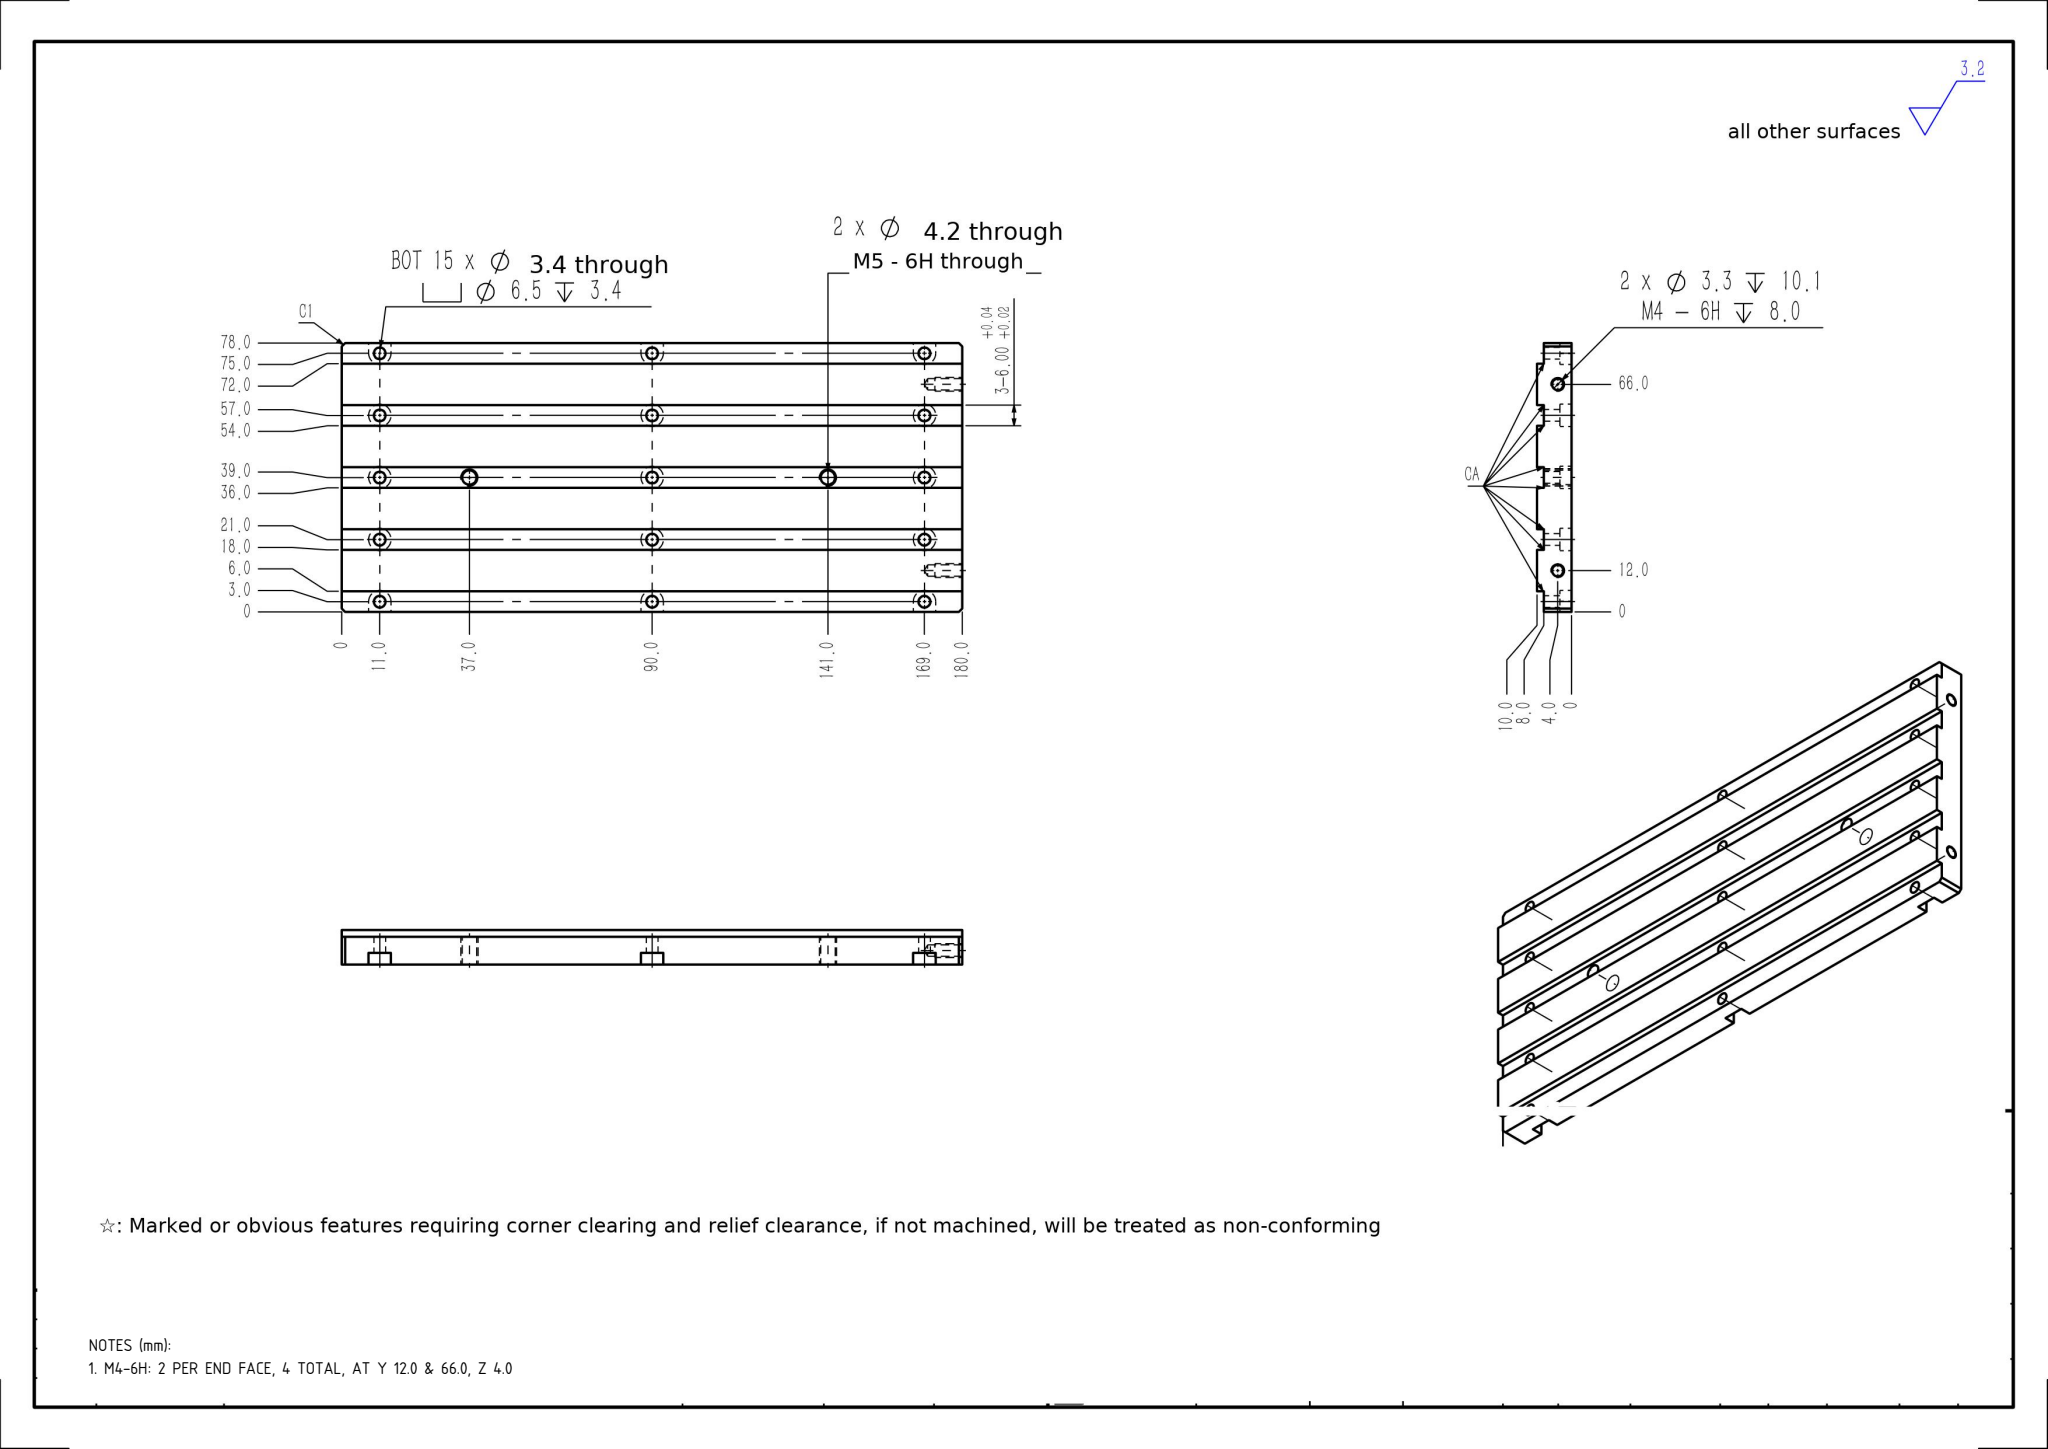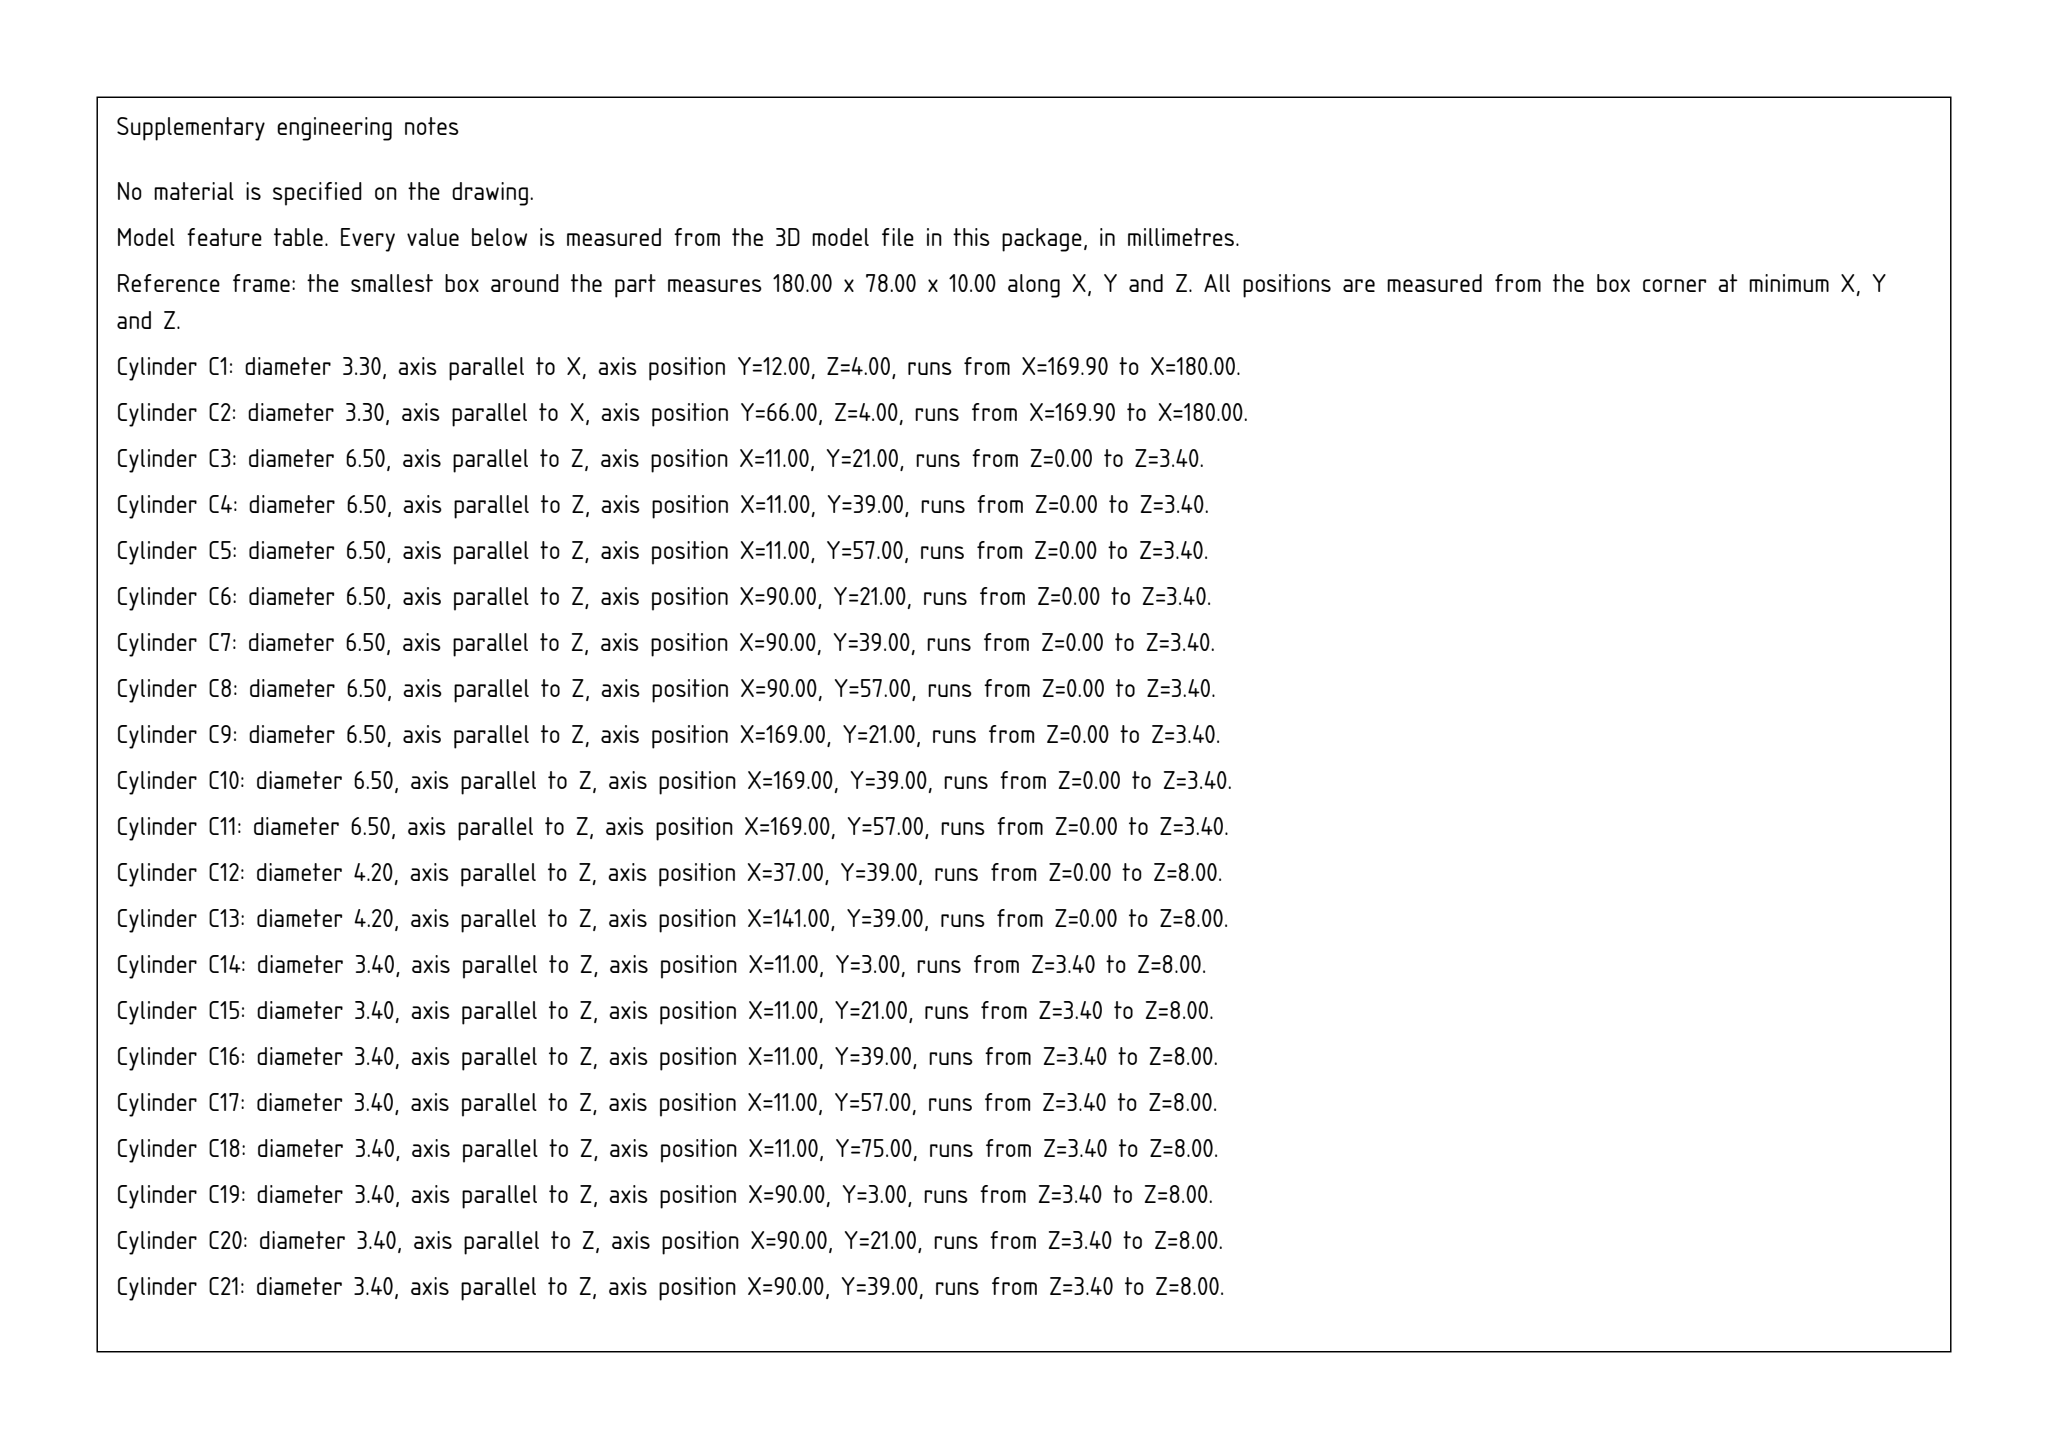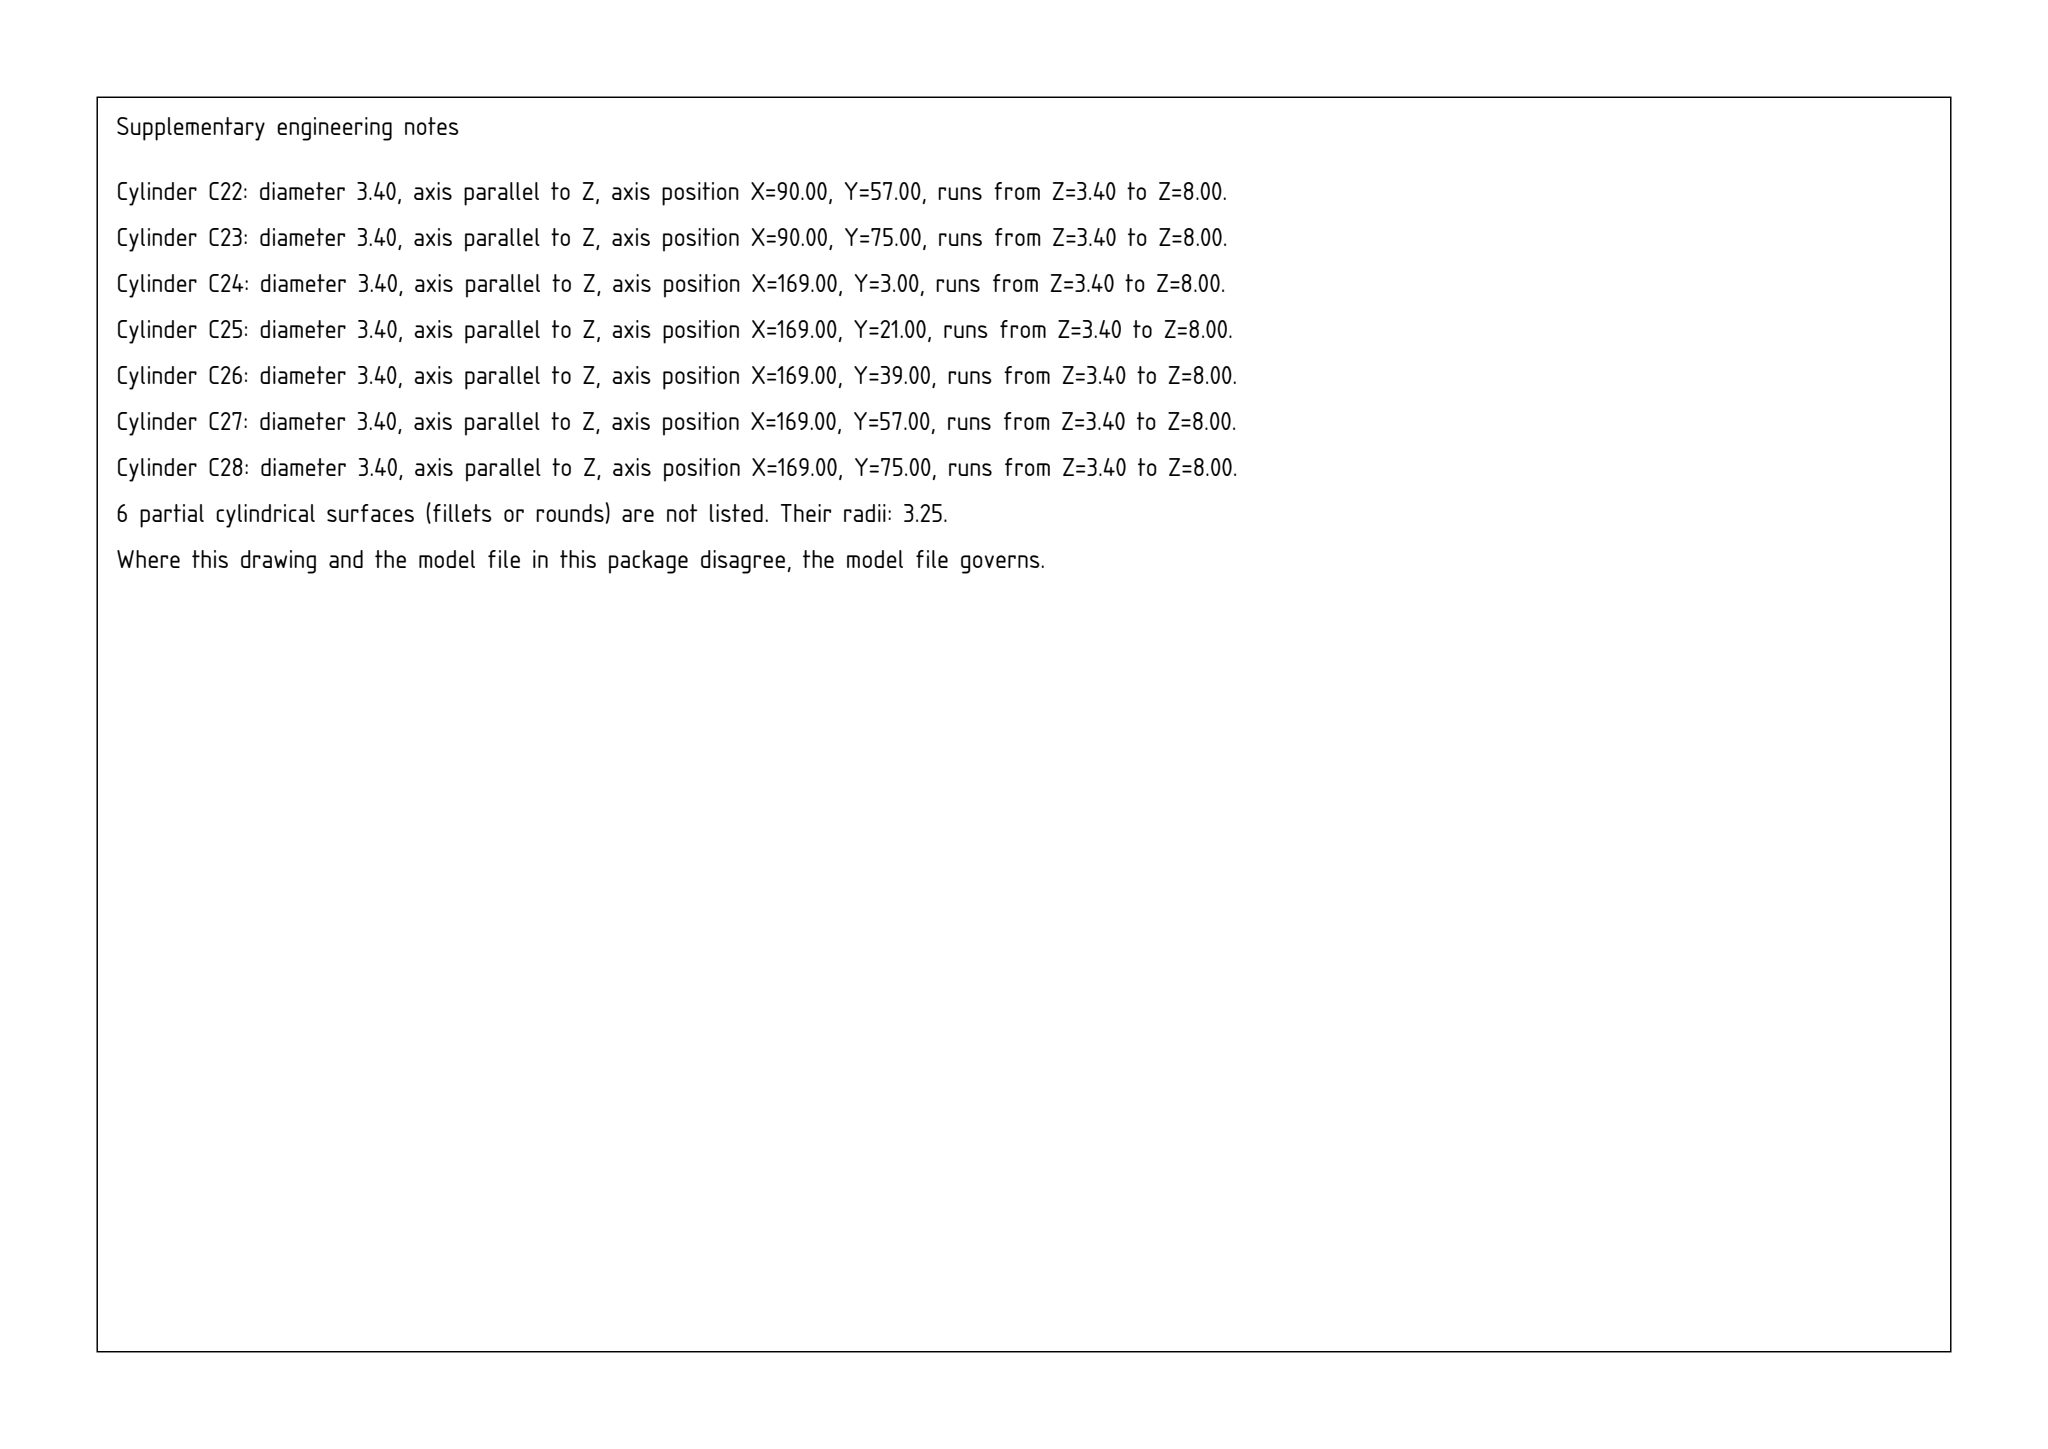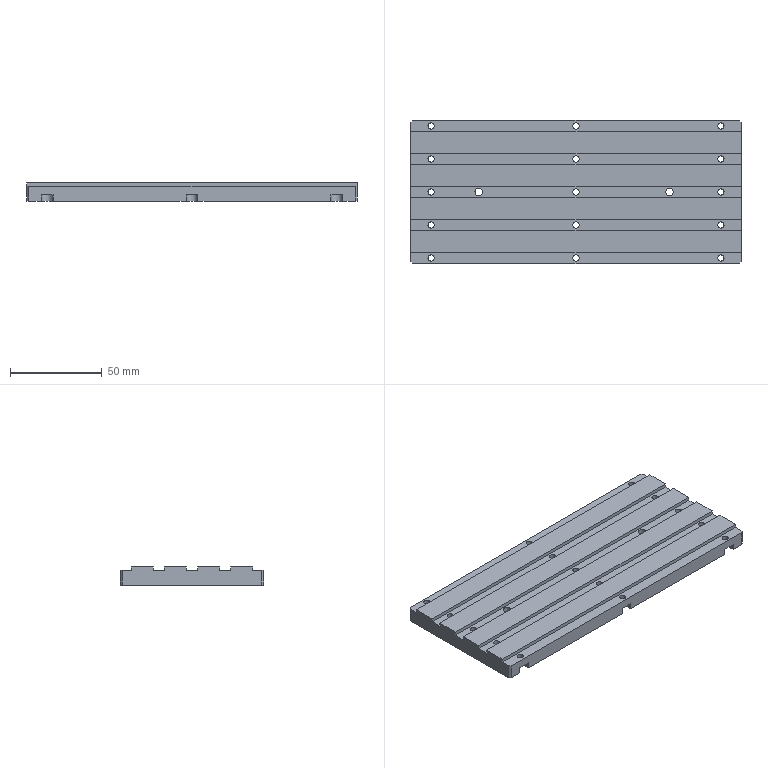Part | SolidWorks | mm | 1 solid | 119 faces | box 180 x 78 x 10 mm | volume 126806 mm3 | cylinder 62 | plane 53 | cone 4 | commonest cylinder face diameters 3.4 x30 6.5 x24 4.2 x4 3.3 x4
Drawing notes:
M4-6H: 2 PER END FACE, 4 TOTAL, AT Y 12.0 & 66.0, Z 4.0 | from the solid: Ø3.3 x-axis cyls, len 10.1, at (y12.0,z4.0) count 2 and (y66.0,z4.0) count 2; bbox x 0-180, end faces x=0 & x=180
build123d program:
from build123d import *

# Parameters (mm, degrees)
SKETCH1_W                                       = 180
SKETCH1_H                                       = 78
BOSS_EXTRUDE1_DEPTH                             = 5
SKETCH2_W                                       = 180
SKETCH2_H                                       = 6
CUT_EXTRUDE1_DEPTH                              = 2
M3_HEX_SOCKET_HEAD_CAP_SCREW_CBORE1_D           = 3.4
M3_HEX_SOCKET_HEAD_CAP_SCREW_CBORE1_CBORE_D     = 6.5
M3_HEX_SOCKET_HEAD_CAP_SCREW_CBORE1_CBORE_DEPTH = 3.4
SKETCH8_W                                       = 6.5
SKETCH8_H                                       = 3
CUT_EXTRUDE2_DEPTH                              = 3.4
CHAMFER1_SIZE                                   = 1
M4_TAPPED_HOLE1_D                               = 3.3
M4_TAPPED_HOLE1_DEPTH                           = 10.1
M4_TAPPED_HOLE1_TIP                             = 0.9914
M5_TAPPED_HOLE1_D                               = 4.2


with BuildPart() as part:
    # Sketch1 → Boss-Extrude1 (new, symmetric)
    with BuildSketch(Plane.XY):
        Rectangle(SKETCH1_W, SKETCH1_H)
    extrude(amount=BOSS_EXTRUDE1_DEPTH, both=True)

    # Sketch2 → Cut-Extrude1 (cut)
    with BuildSketch(Plane.XY.offset(5)):
        with Locations((0, -36)):
            Rectangle(SKETCH2_W, SKETCH2_H)
        with Locations((0, -18)):
            Rectangle(SKETCH2_W, SKETCH2_H)
        Rectangle(SKETCH2_W, SKETCH2_H)
        with Locations((0, 18)):
            Rectangle(SKETCH2_W, SKETCH2_H)
        with Locations((0, 36)):
            Rectangle(SKETCH2_W, SKETCH2_H)
    extrude(amount=-CUT_EXTRUDE1_DEPTH, mode=Mode.SUBTRACT)

    # M3 Hex Socket Head Cap Screw CBORE1 (through all)
    with Locations(Plane(origin=(0, 0, -5), x_dir=(-1, 0, 0), z_dir=(0, 0, -1))):
        with Locations((79, -36), (0, -36), (-79, -36), (79, -18), (0, -18), (-79, -18), (79, 0), (0, 0), (-79, 0), (79, 18), (0, 18), (-79, 18), (79, 36), (0, 36), (-79, 36)):
            CounterBoreHole(M3_HEX_SOCKET_HEAD_CAP_SCREW_CBORE1_D / 2, M3_HEX_SOCKET_HEAD_CAP_SCREW_CBORE1_CBORE_D / 2, M3_HEX_SOCKET_HEAD_CAP_SCREW_CBORE1_CBORE_DEPTH)

    # Sketch8 → Cut-Extrude2 (cut)
    with BuildSketch(Plane(origin=(0, 0, -5), x_dir=(-1, 0, 0), z_dir=(0, 0, -1))):
        with Locations((-79, 37.5)):
            Rectangle(SKETCH8_W, SKETCH8_H)
        with Locations((0, 37.5)):
            Rectangle(SKETCH8_W, SKETCH8_H)
        with Locations((79, 37.5)):
            Rectangle(SKETCH8_W, SKETCH8_H)
        with Locations((-79, -37.5)):
            Rectangle(SKETCH8_W, SKETCH8_H)
        with Locations((0, -37.5)):
            Rectangle(SKETCH8_W, SKETCH8_H)
        with Locations((79, -37.5)):
            Rectangle(SKETCH8_W, SKETCH8_H)
    extrude(amount=-CUT_EXTRUDE2_DEPTH, mode=Mode.SUBTRACT)

    # Chamfer1
    chamfer1_edges = [part.edges().sort_by_distance(p)[0] for p in [
        (90, -39, -1),
        (-90, -39, -1),
        (-90, 39, -1),
        (90, 39, -1),
    ]]
    chamfer(chamfer1_edges, length=CHAMFER1_SIZE)

    # M4 Tapped Hole1
    with Locations(Plane(origin=(90, 0, 0), x_dir=(0, 0, -1), z_dir=(1, 0, 0))):
        with Locations((1, 27), (1, -27)):
            Hole(M4_TAPPED_HOLE1_D / 2, depth=M4_TAPPED_HOLE1_DEPTH)
            with Locations((0, 0, -(M4_TAPPED_HOLE1_DEPTH + M4_TAPPED_HOLE1_TIP / 2))):  # 118° drill point
                Cone(0, M4_TAPPED_HOLE1_D / 2, M4_TAPPED_HOLE1_TIP, mode=Mode.SUBTRACT)

    # M5 Tapped Hole1 (through all)
    with Locations(Plane(origin=(0, 0, -5), x_dir=(-1, 0, 0), z_dir=(0, 0, -1))):
        with Locations((53, 0), (-51, 0)):
            Hole(M5_TAPPED_HOLE1_D / 2)


solid = part.part